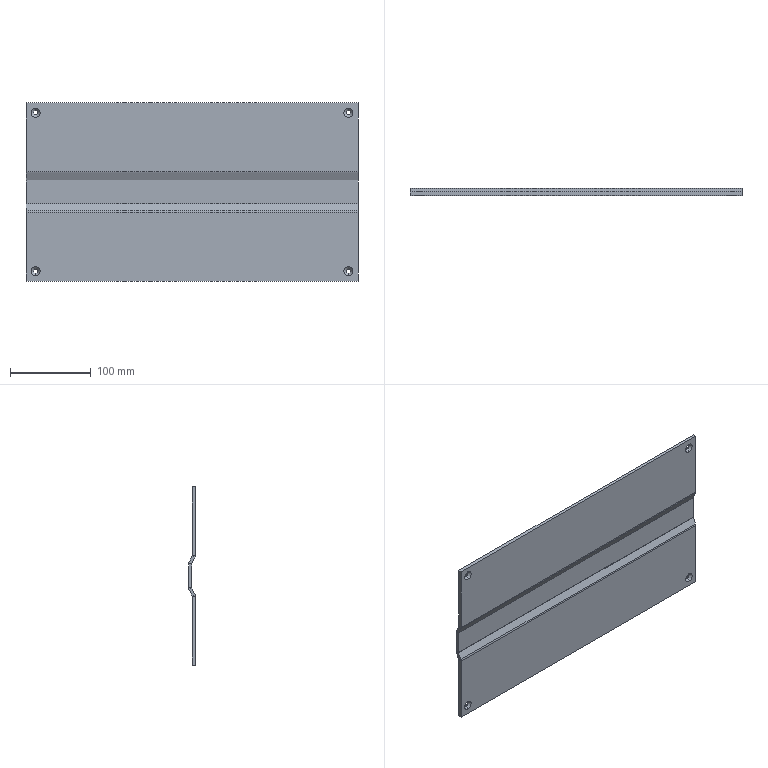Component | SolidWorks | Q1-A12-S21-Q4-02A-4 | 1 solid | 54 faces | volume 363153 mm3 | plane 30 | cylinder 16 | cone 8 | commonest cylinder face diameters 5.5 x8 9.473 x4 1.473 x4 | material SUS-304